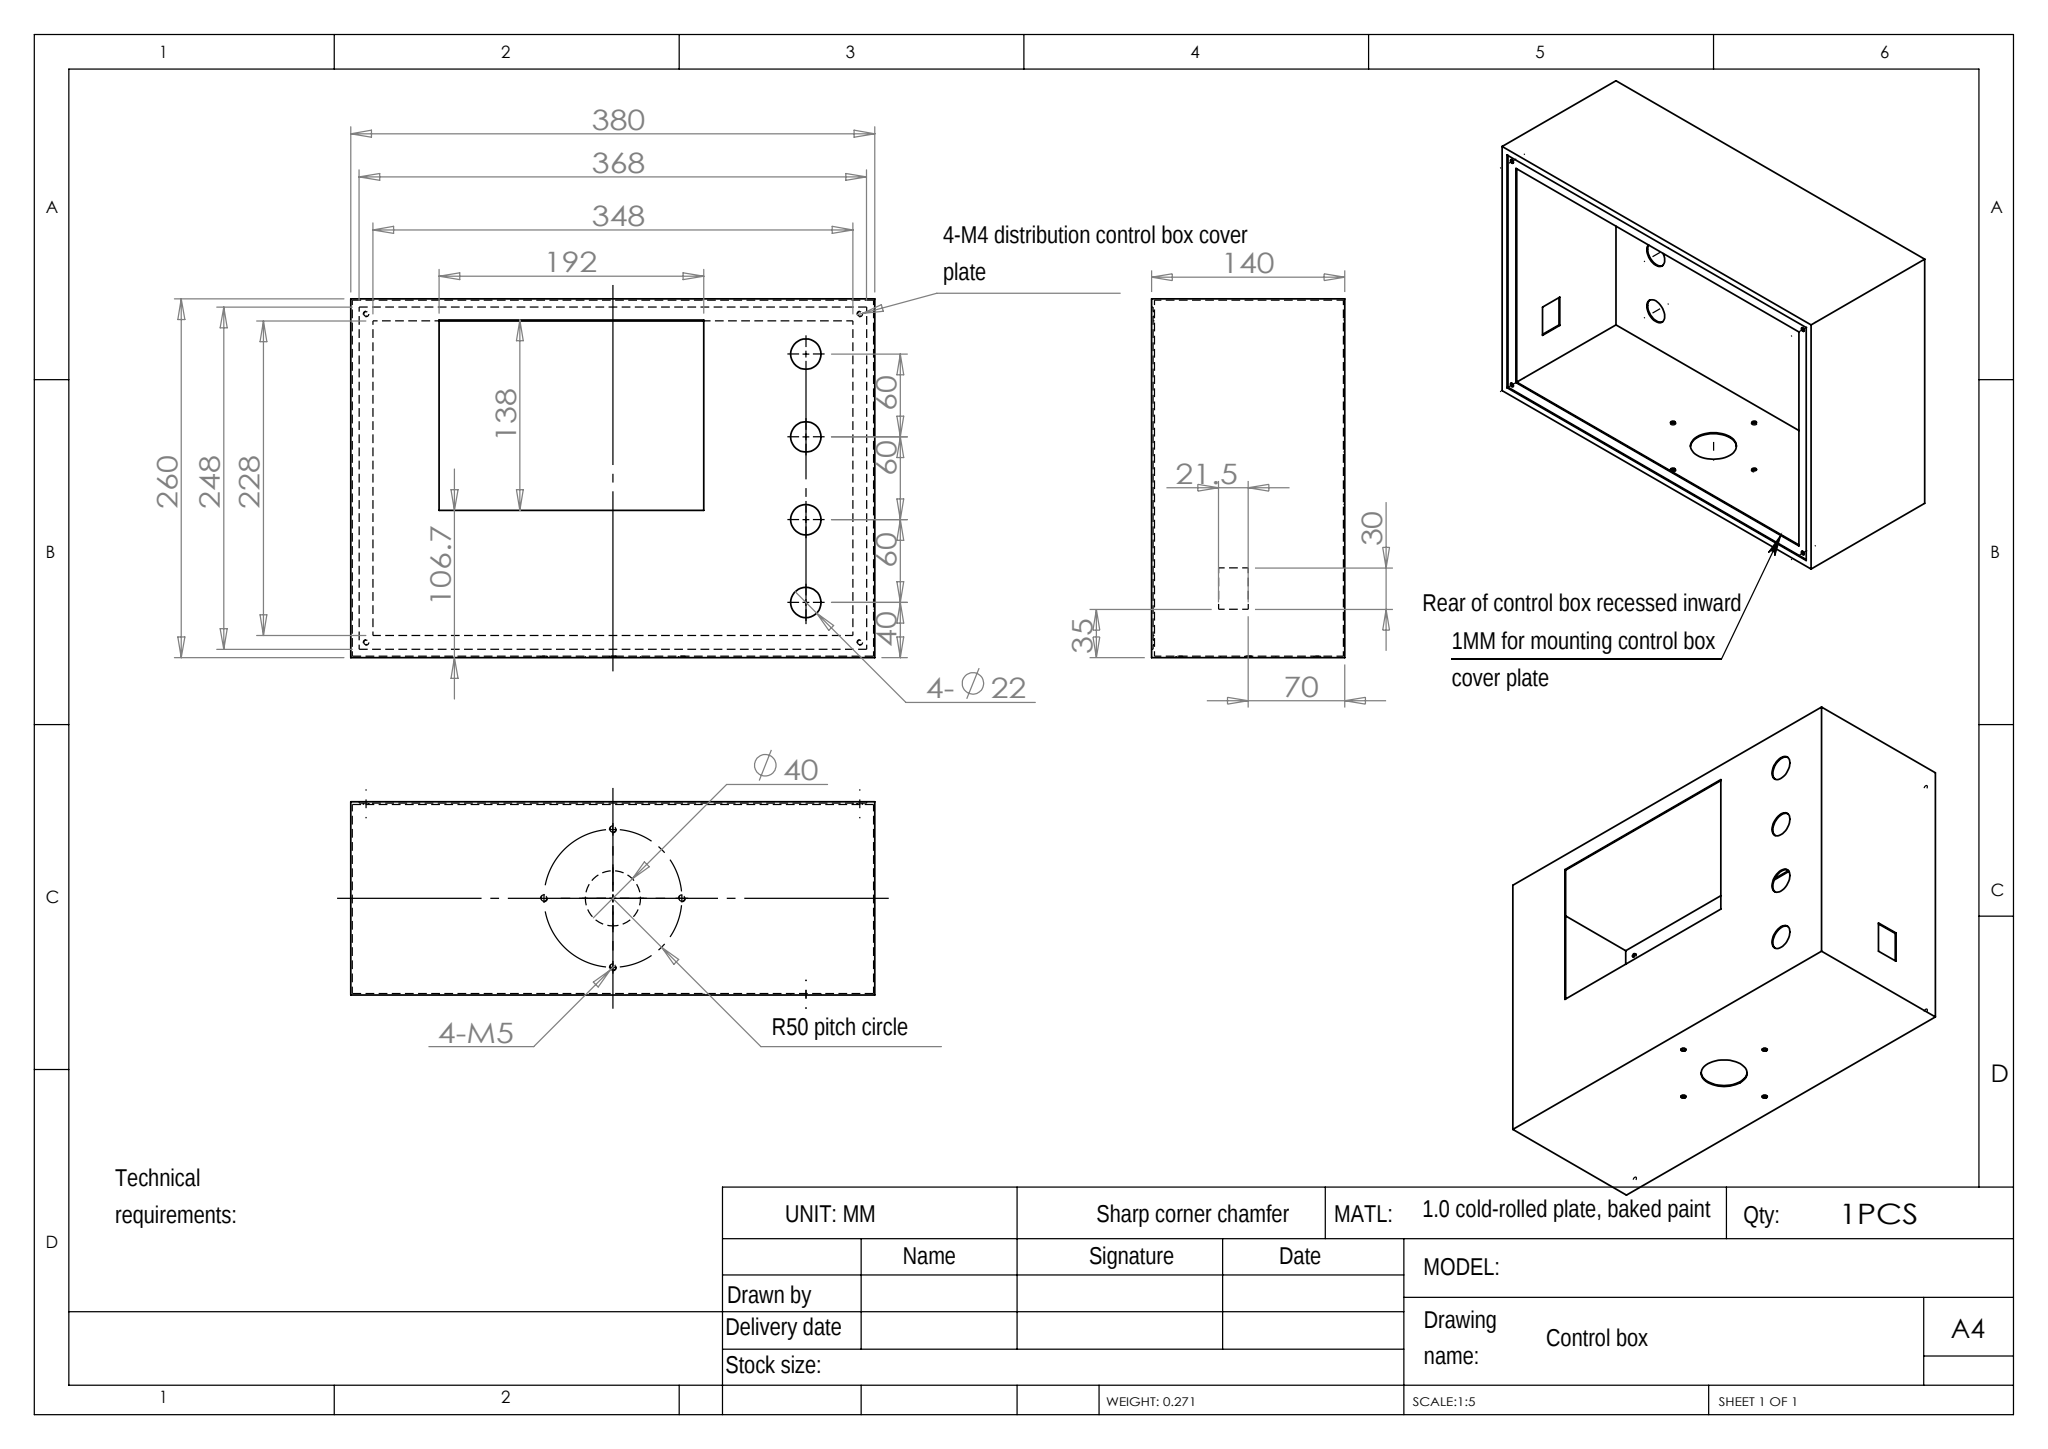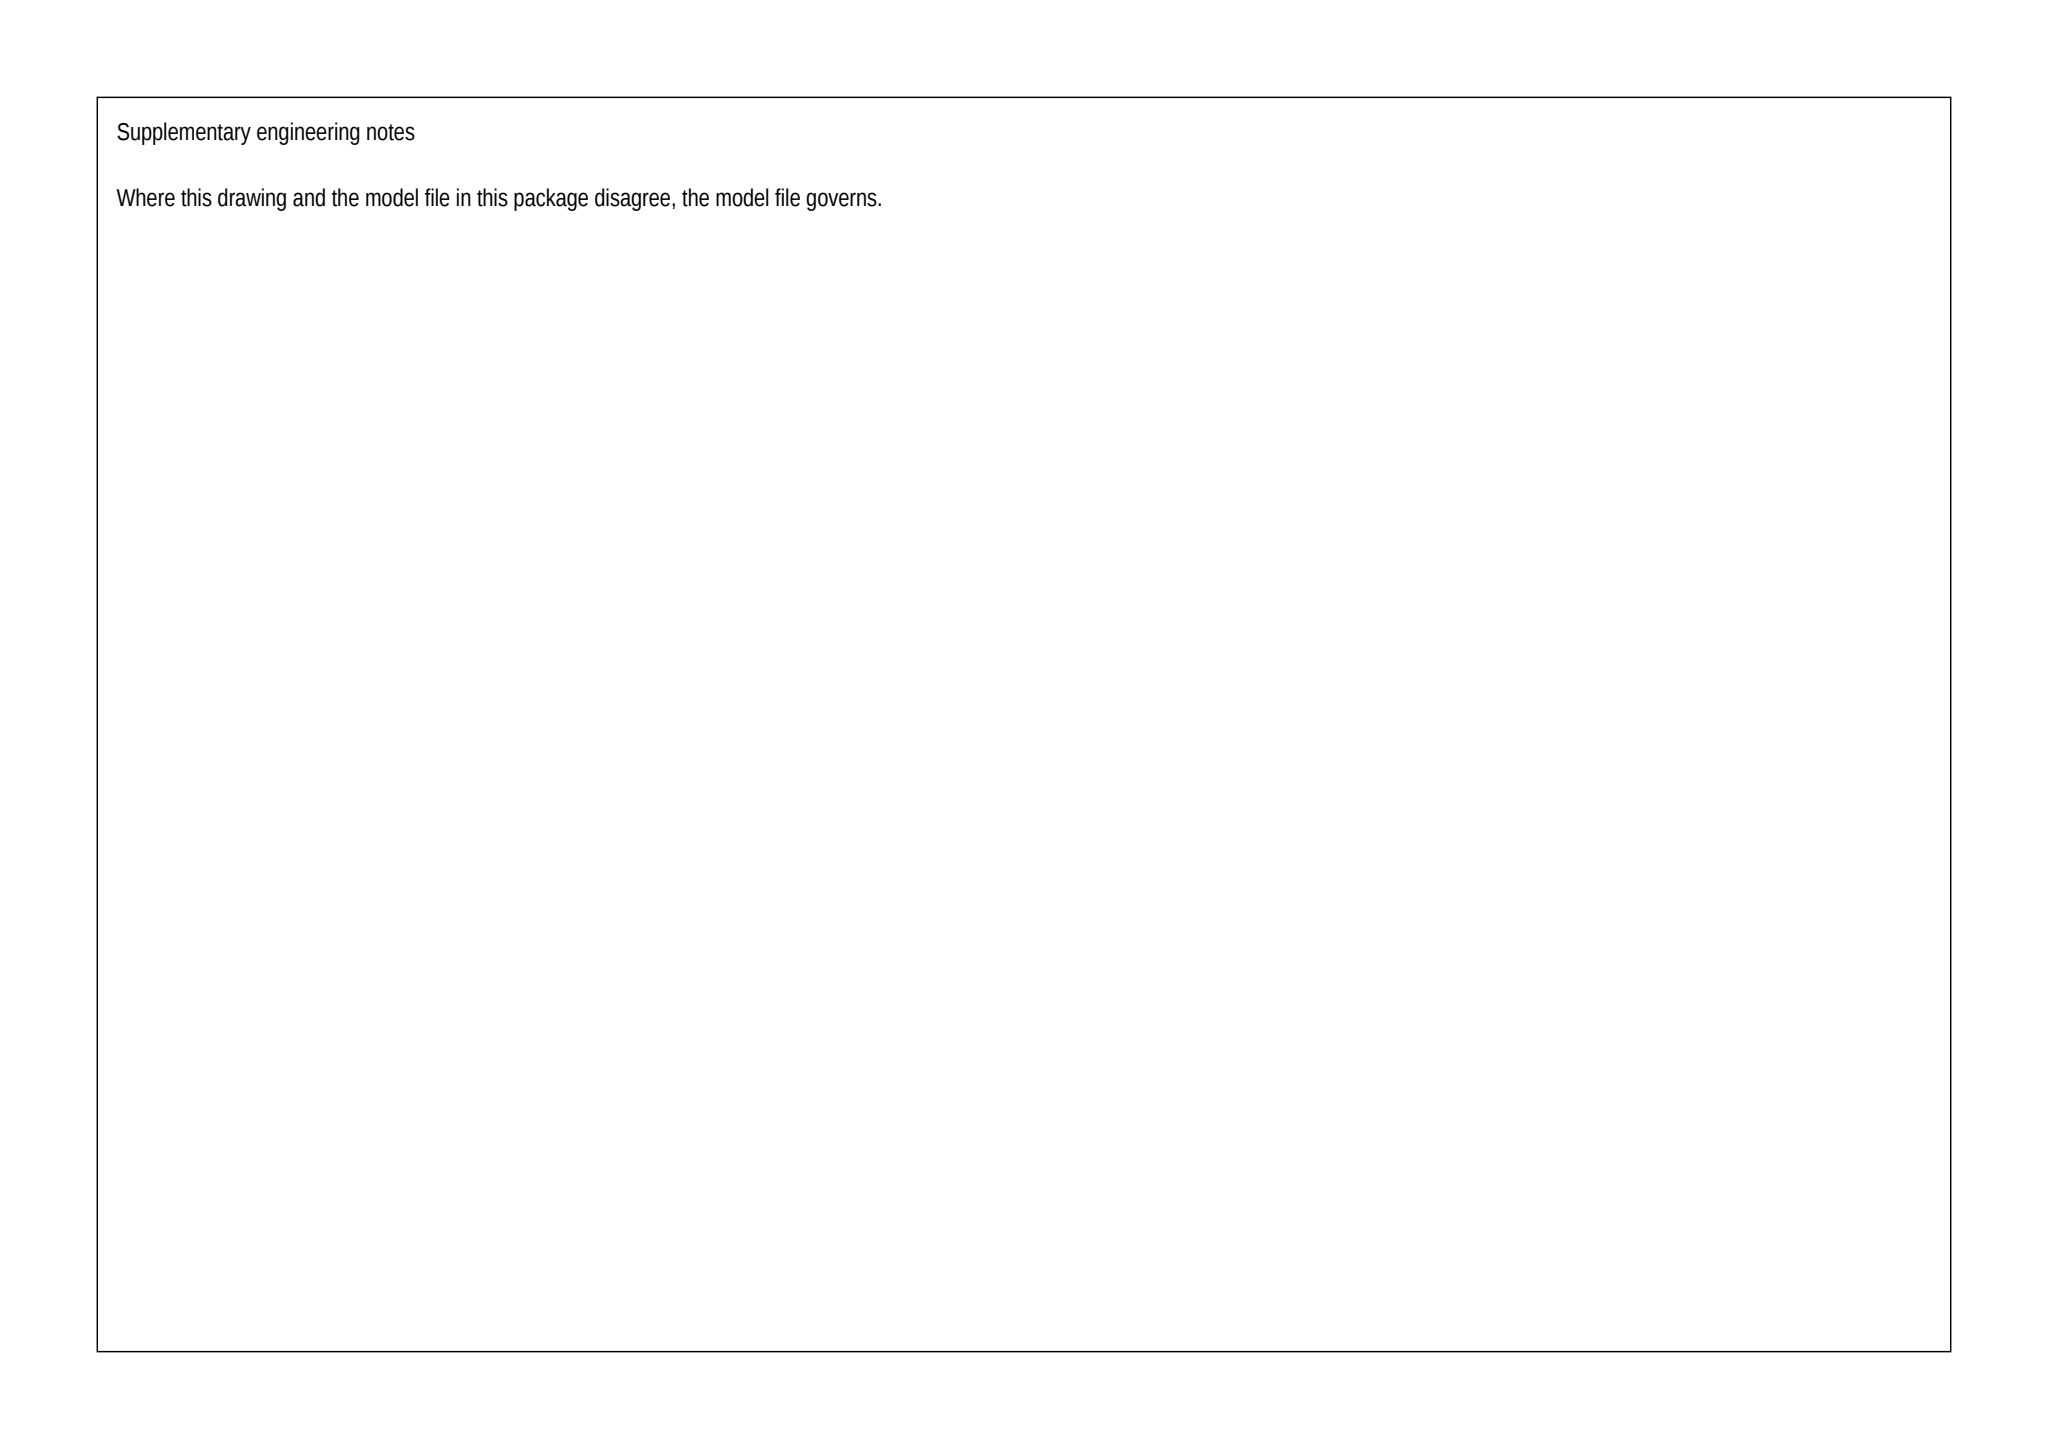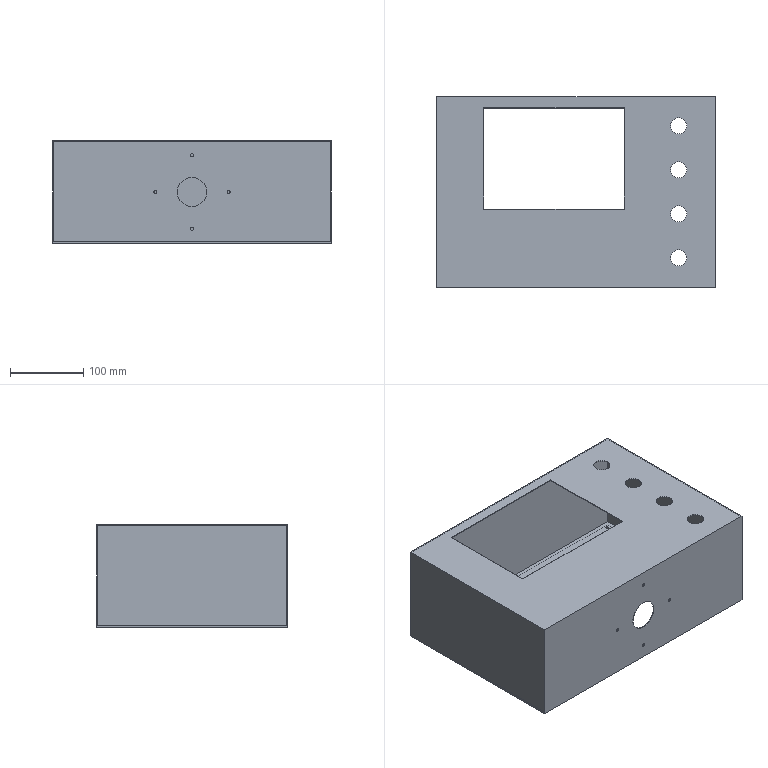Part | SolidWorks | mm | material 1.0 Cold-rolled sheet, painted | 1 solid | 55 faces | box 380 x 260 x 140 mm | volume 270596 mm3 | plane 29 | cylinder 26 | commonest cylinder face diameters 4.2 x8 22 x8 3.3 x8 40 x2
Drawing notes:
FRONT VIEW: 64 FROM LH EDGE TO WINDOW CUTOUT 192 x 138 | from the solid: Planes x=64 & x=256, y=106.7 & y=244.7 at z=139-140: cutout 192 wide x 138 high, left edge 64 from x=0
4-M4 ON REAR FLANGE: 11 FROM EACH EDGE, 358 x 238 PITCH | from the solid: Ø3.3 holes, axis z, at (11,11),(11,249),(369,11),(369,249), z=1 to 2
4-Ø22 CL 50 FROM RH EDGE, LOWEST 40 FROM BOT, 60 PITCH | from the solid: Ø22 holes axis z at x=330 (380-330=50), y=40,100,160,220, z=139-140
4-M4 FOR REAR COVER PLATE; BOX DEPTH 140 | from the solid: bbox_xyz z extent = 140; Ø3.3 (M4) holes at recessed rear face z=1-2
build123d program:
from build123d import *

# Parameters (mm, degrees)
SKETCH1_W             = 380
SKETCH1_H             = 260
BOSS_EXTRUDE1_DEPTH   = 140
SHELL1_T              = -1
SKETCH2_W             = 380
SKETCH2_H             = 260
BOSS_EXTRUDE2_DEPTH   = 2
SKETCH3_W             = 368
SKETCH3_H             = 248
CUT_EXTRUDE1_DEPTH    = 1
SKETCH4_W             = 348
SKETCH4_H             = 228
CUT_EXTRUDE2_DEPTH    = 1
M4_TAPPED_HOLE1_D     = 3.3
M4_TAPPED_HOLE1_DEPTH = 11.5
M4_TAPPED_HOLE1_TIP   = 0.9914
SKETCH8_W             = 192
SKETCH8_H             = 138
CUT_EXTRUDE3_DEPTH    = 1
SKETCH9_R             = 11
CUT_EXTRUDE4_DEPTH    = 10
SKETCH10_R            = 20
CUT_EXTRUDE5_DEPTH    = 10
SKETCH11_W            = 21.5
SKETCH11_H            = 30
CUT_EXTRUDE6_DEPTH    = 10
CIRPATTERN1_COUNT     = 4


with BuildPart() as part:
    # Sketch1 → Boss-Extrude1 (new body)
    with BuildSketch(Plane.XY):
        with Locations((190, -130)):
            Rectangle(SKETCH1_W, SKETCH1_H)
    extrude(amount=BOSS_EXTRUDE1_DEPTH)

    # Shell1
    shell1_openings = [part.faces().sort_by_distance(p)[0] for p in [
        (190, -130, 0),
    ]]
    offset(amount=SHELL1_T, openings=shell1_openings, kind=Kind.INTERSECTION)

    # Sketch2 → Boss-Extrude2 (add)
    with BuildSketch(Plane(origin=(0, 0, 0), x_dir=(-1, 0, 0), z_dir=(0, 0, -1))):
        with Locations((-190, -130)):
            Rectangle(SKETCH2_W, SKETCH2_H)
    extrude(amount=-BOSS_EXTRUDE2_DEPTH)

    # Sketch3 → Cut-Extrude1 (cut)
    with BuildSketch(Plane(origin=(0, 0, 0), x_dir=(-1, 0, 0), z_dir=(0, 0, -1))):
        with Locations((-190, -130)):
            Rectangle(SKETCH3_W, SKETCH3_H)
    extrude(amount=-CUT_EXTRUDE1_DEPTH, mode=Mode.SUBTRACT)

    # Sketch4 → Cut-Extrude2 (cut)
    with BuildSketch(Plane(origin=(0, 0, 1), x_dir=(-1, 0, 0), z_dir=(0, 0, -1))):
        with Locations((-190, -130)):
            Rectangle(SKETCH4_W, SKETCH4_H)
    extrude(amount=-CUT_EXTRUDE2_DEPTH, mode=Mode.SUBTRACT)

    # M4 Tapped Hole1
    with Locations(Plane(origin=(0, 0, 1), x_dir=(-1, 0, 0), z_dir=(0, 0, -1))):
        with Locations((-369, -11), (-369, -249), (-11, -11), (-11, -249)):
            Hole(M4_TAPPED_HOLE1_D / 2, depth=M4_TAPPED_HOLE1_DEPTH)
            with Locations((0, 0, -(M4_TAPPED_HOLE1_DEPTH + M4_TAPPED_HOLE1_TIP / 2))):  # 118° drill point
                Cone(0, M4_TAPPED_HOLE1_D / 2, M4_TAPPED_HOLE1_TIP, mode=Mode.SUBTRACT)

    # Sketch8 → Cut-Extrude3 (cut)
    with BuildSketch(Plane.XY.offset(140)):
        with Locations((160, -84.334)):
            Rectangle(SKETCH8_W, SKETCH8_H)
    extrude(amount=-CUT_EXTRUDE3_DEPTH, mode=Mode.SUBTRACT)

    # Sketch9 → Cut-Extrude4 (cut)
    with BuildSketch(Plane.XY.offset(140)):
        with Locations((330, -160)):
            Circle(SKETCH9_R)
        with Locations((330, -220)):
            Circle(SKETCH9_R)
        with Locations((330, -100)):
            Circle(SKETCH9_R)
        with Locations((330, -40)):
            Circle(SKETCH9_R)
    extrude(amount=-CUT_EXTRUDE4_DEPTH, mode=Mode.SUBTRACT)

    # Sketch10 → Cut-Extrude5 (cut)
    with BuildSketch(Plane.XZ.offset(260)):
        with Locations(Location((190, 70, 0), (0, 0, 270))):
            Circle(SKETCH10_R)
    extrude(amount=-CUT_EXTRUDE5_DEPTH, mode=Mode.SUBTRACT)

    # Sketch11 → Cut-Extrude6 (cut)
    with BuildSketch(Plane(origin=(380, 0, 0), x_dir=(0, 0, -1), z_dir=(1, 0, 0))):
        with Locations((-59.25, -210)):
            Rectangle(SKETCH11_W, SKETCH11_H)
    extrude(amount=-CUT_EXTRUDE6_DEPTH, mode=Mode.SUBTRACT)

    # Sketch12 → M5 Tapped Hole1 (revolve, cut)
    with BuildSketch(Plane(origin=(190, -260, 120), x_dir=(0, 0, -1), z_dir=(1, 0, 0))):
        Polygon((0, 0), (0, 15.262), (2.1, 14), (2.1, 0), align=None)
    m5_tapped_hole1 = revolve(axis=Axis((190, -266.35, 120), (0, 1, 0)), mode=Mode.SUBTRACT)

    # CirPattern1: M5 Tapped Hole1 ×4 about axis
    cirpattern1_axis = Axis((190, 0, 70), (0, 1, 0))
    for i in range(1, CIRPATTERN1_COUNT):
        add(m5_tapped_hole1.rotate(cirpattern1_axis, i * 360 / CIRPATTERN1_COUNT), mode=Mode.SUBTRACT)


solid = part.part